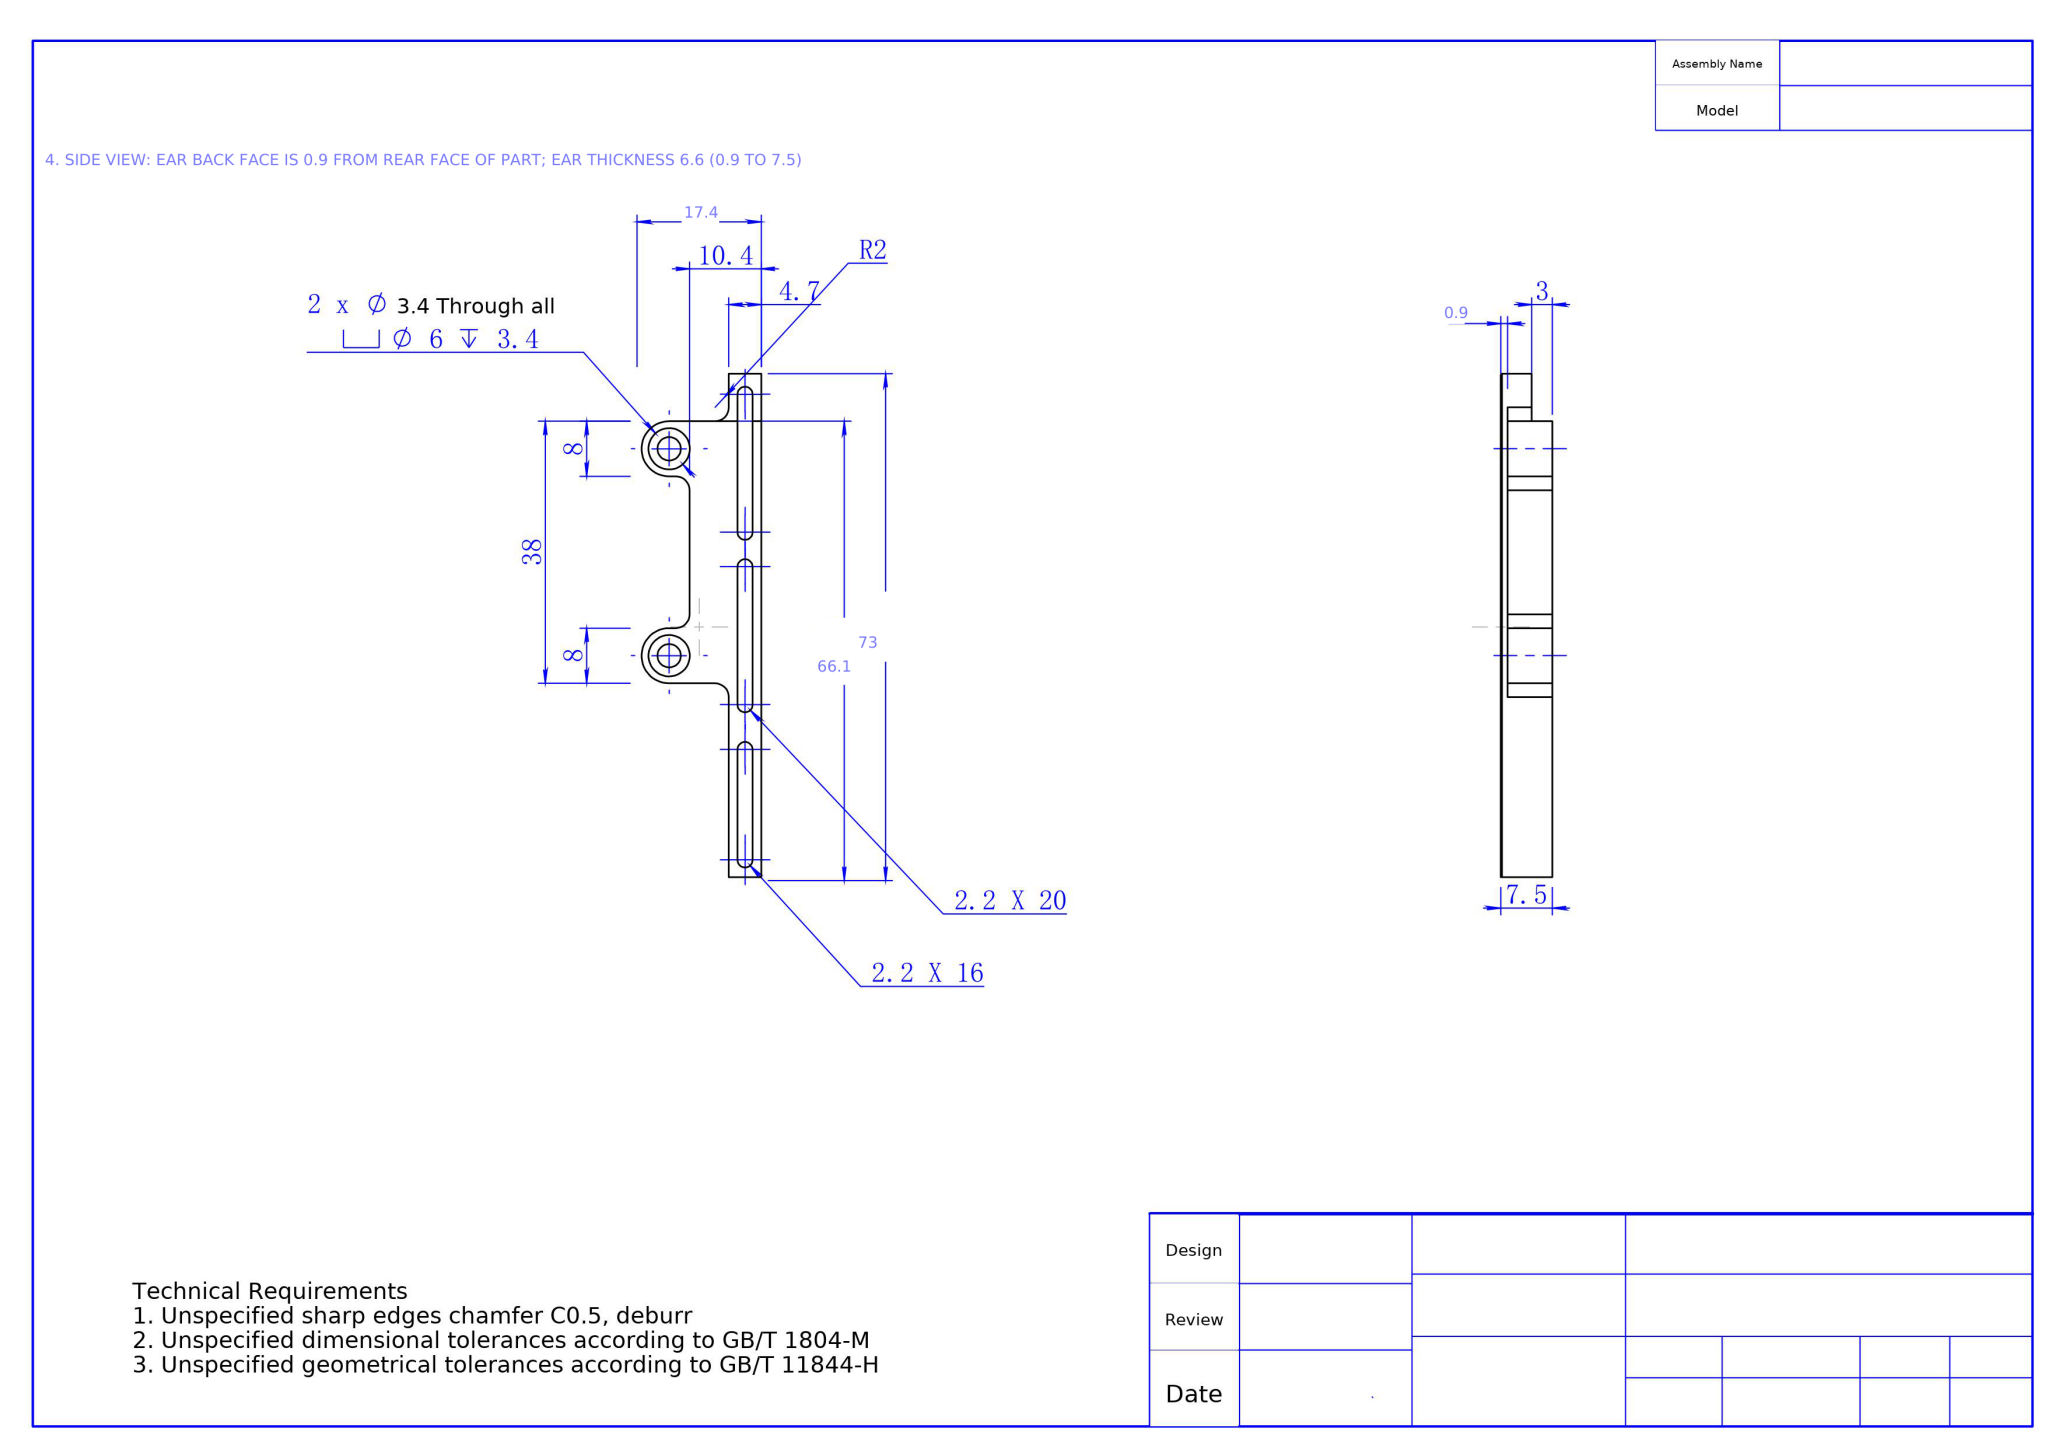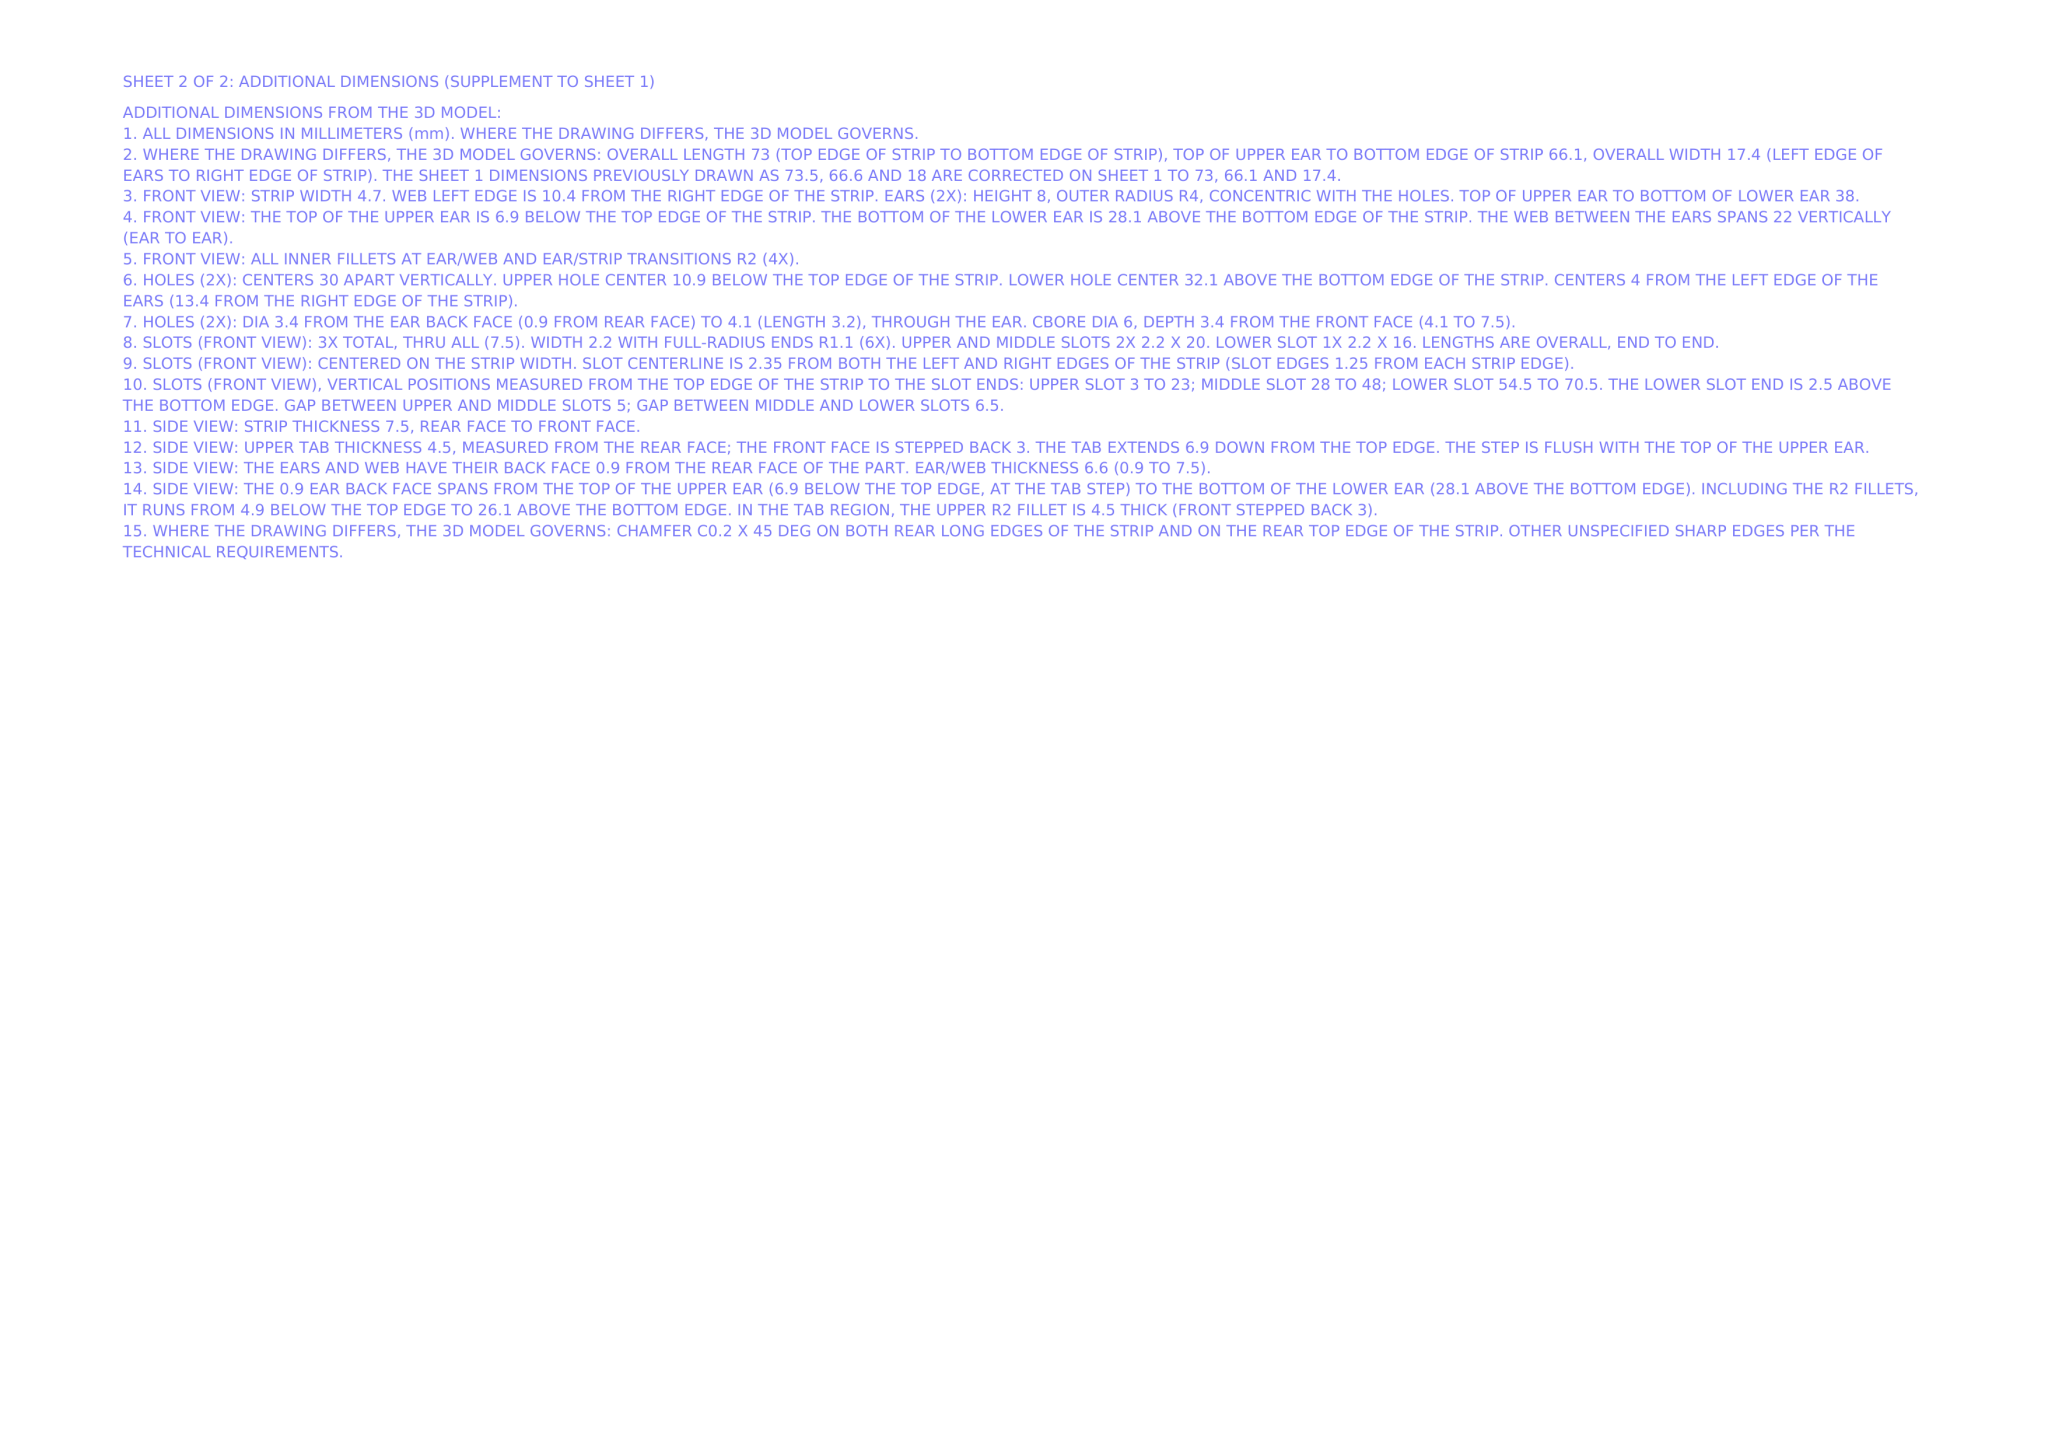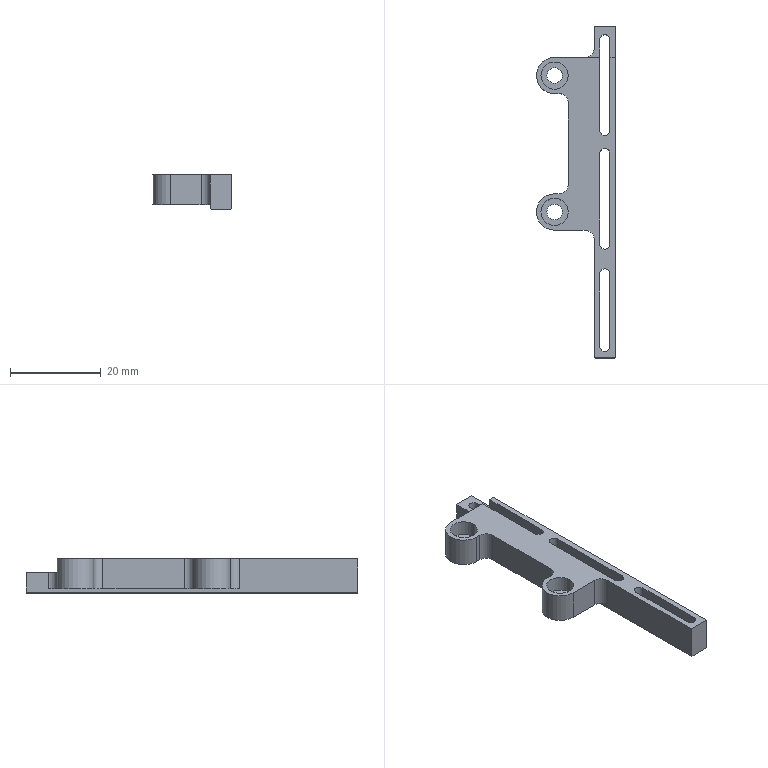Part | NX | mm | 1 solid | 45 faces | box 17.4 x 73 x 7.5 mm | volume 3343 mm3 | plane 25 | cylinder 20 | commonest cylinder face diameters 2.2 x6 6 x4 3.4 x4 4 x4 8 x2